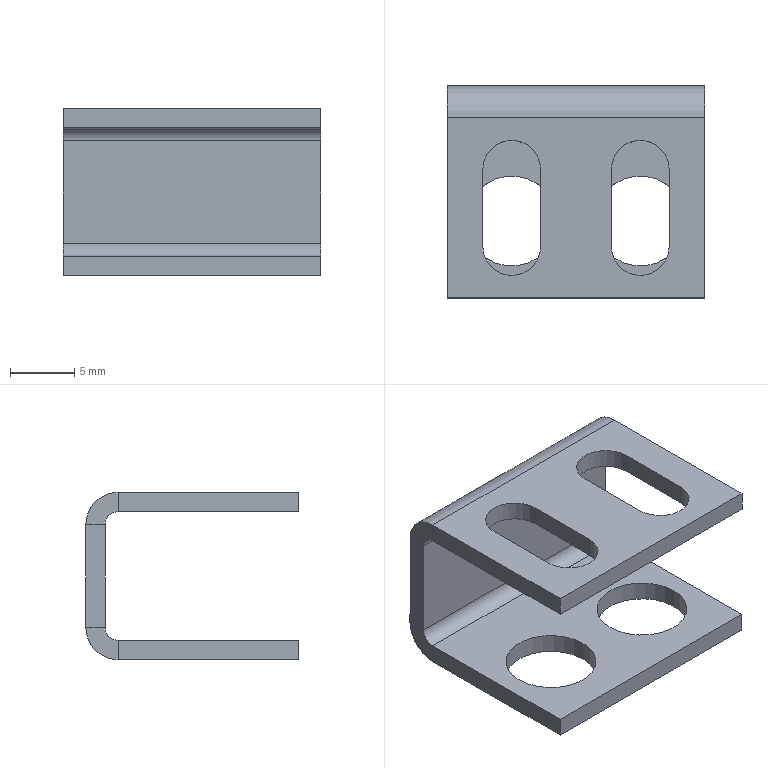Component | SolidWorks | ZSensorPiece-1 | 1 solid | 34 faces | volume 1001 mm3 | plane 22 | cylinder 12 | commonest cylinder face diameters 7 x4 4.5 x4 5 x2 2 x2